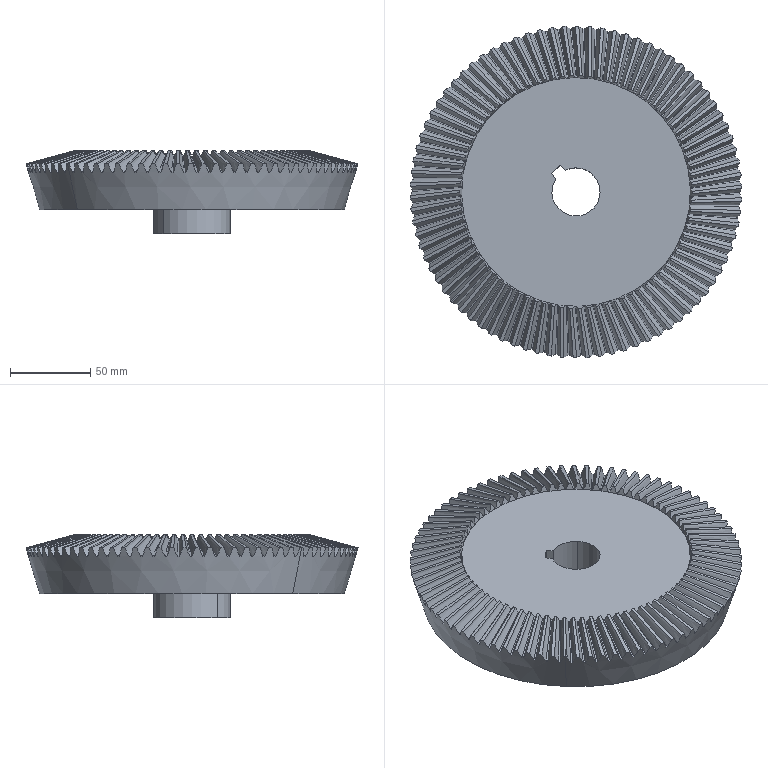Component | SolidWorks | BevelGear82_2.51-1 | 1 solid | 344 faces | volume 973087 mm3 | spline 246 | cone 87 | plane 6 | cylinder 5 | commonest cylinder face diameters 30 x3 48 x2